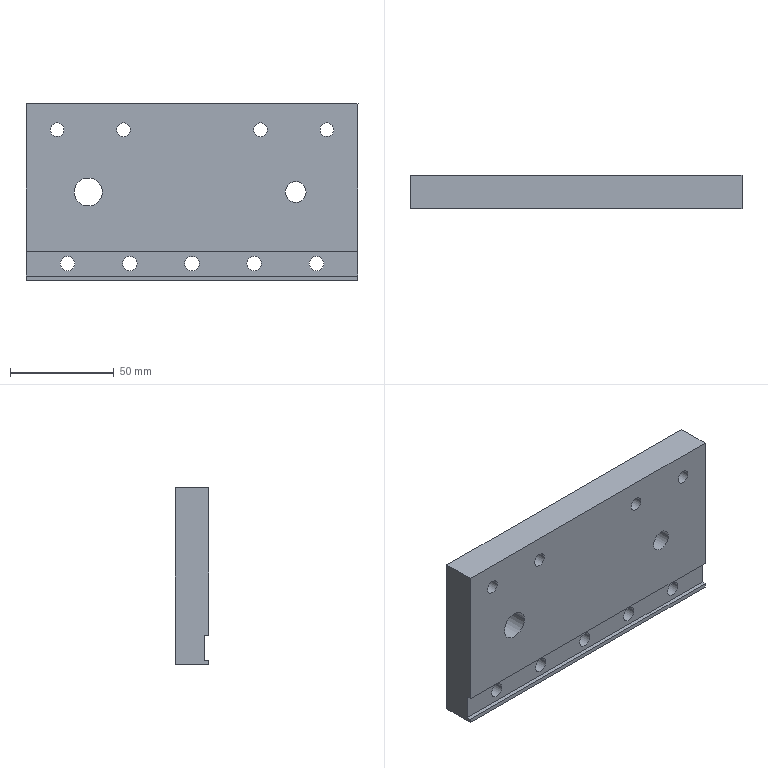Component | SolidWorks | BevelGearPlate1-2 | 1 solid | 44 faces | box 160 x 16 x 85 mm | volume 203859 mm3 | cylinder 30 | plane 14 | commonest cylinder face diameters 7 x10 11 x8 6.6 x8 13.532 x2 10 x2
build123d program:
from build123d import *

# Parameters (mm, degrees)
SKETCH1_W                                       = 160
SKETCH1_H                                       = 85
SKETCH1_R                                       = 5
SKETCH1_R_2                                     = 6.766
SKETCH1_R_3                                     = 3.5
EXTRUDE1_DEPTH                                  = 16
SKETCH2_W                                       = 160
SKETCH2_H                                       = 12
EXTRUDE2_DEPTH                                  = 2
M6_HEX_SOCKET_HEAD_CAP_SCREW_CBORE1_D           = 6.6
M6_HEX_SOCKET_HEAD_CAP_SCREW_CBORE1_CBORE_D     = 11
M6_HEX_SOCKET_HEAD_CAP_SCREW_CBORE1_CBORE_DEPTH = 6


with BuildPart() as part:
    # Sketch1 → Extrude1 (new body)
    with BuildSketch(Plane.XY):
        with Locations((17.215, -22.673)):
            Rectangle(SKETCH1_W, SKETCH1_H)
        with Locations((-32.785, -22.673)):
            Circle(SKETCH1_R, mode=Mode.SUBTRACT)
        with Locations((67.215, -22.673)):
            Circle(SKETCH1_R_2, mode=Mode.SUBTRACT)
        with Locations((17.215, 11.827)):
            Circle(SKETCH1_R_3, mode=Mode.SUBTRACT)
        with Locations((47.215, 11.827)):
            Circle(SKETCH1_R_3, mode=Mode.SUBTRACT)
        with Locations((77.215, 11.827)):
            Circle(SKETCH1_R_3, mode=Mode.SUBTRACT)
        with Locations((-12.785, 11.827)):
            Circle(SKETCH1_R_3, mode=Mode.SUBTRACT)
        with Locations((-42.785, 11.827)):
            Circle(SKETCH1_R_3, mode=Mode.SUBTRACT)
    extrude(amount=EXTRUDE1_DEPTH)

    # Sketch2 → Extrude2 (cut)
    with BuildSketch(Plane.XY.offset(16)):
        with Locations((17.215, 11.827)):
            Rectangle(SKETCH2_W, SKETCH2_H)
    extrude(amount=-EXTRUDE2_DEPTH, mode=Mode.SUBTRACT)

    # M6 Hex Socket Head Cap Screw CBORE1 (through all)
    with Locations(Plane(origin=(0, 0, 0), x_dir=(-1, 0, 0), z_dir=(0, 0, -1))):
        with Locations((47.785, -52.673), (15.785, -52.673), (-50.215, -52.673), (-82.215, -52.673)):
            CounterBoreHole(M6_HEX_SOCKET_HEAD_CAP_SCREW_CBORE1_D / 2, M6_HEX_SOCKET_HEAD_CAP_SCREW_CBORE1_CBORE_D / 2, M6_HEX_SOCKET_HEAD_CAP_SCREW_CBORE1_CBORE_DEPTH)


solid = part.part

# Placed as in the assembly
solid = solid.moved(Location((-175.406, 628.983, -132.389), (90, 0, -180)))